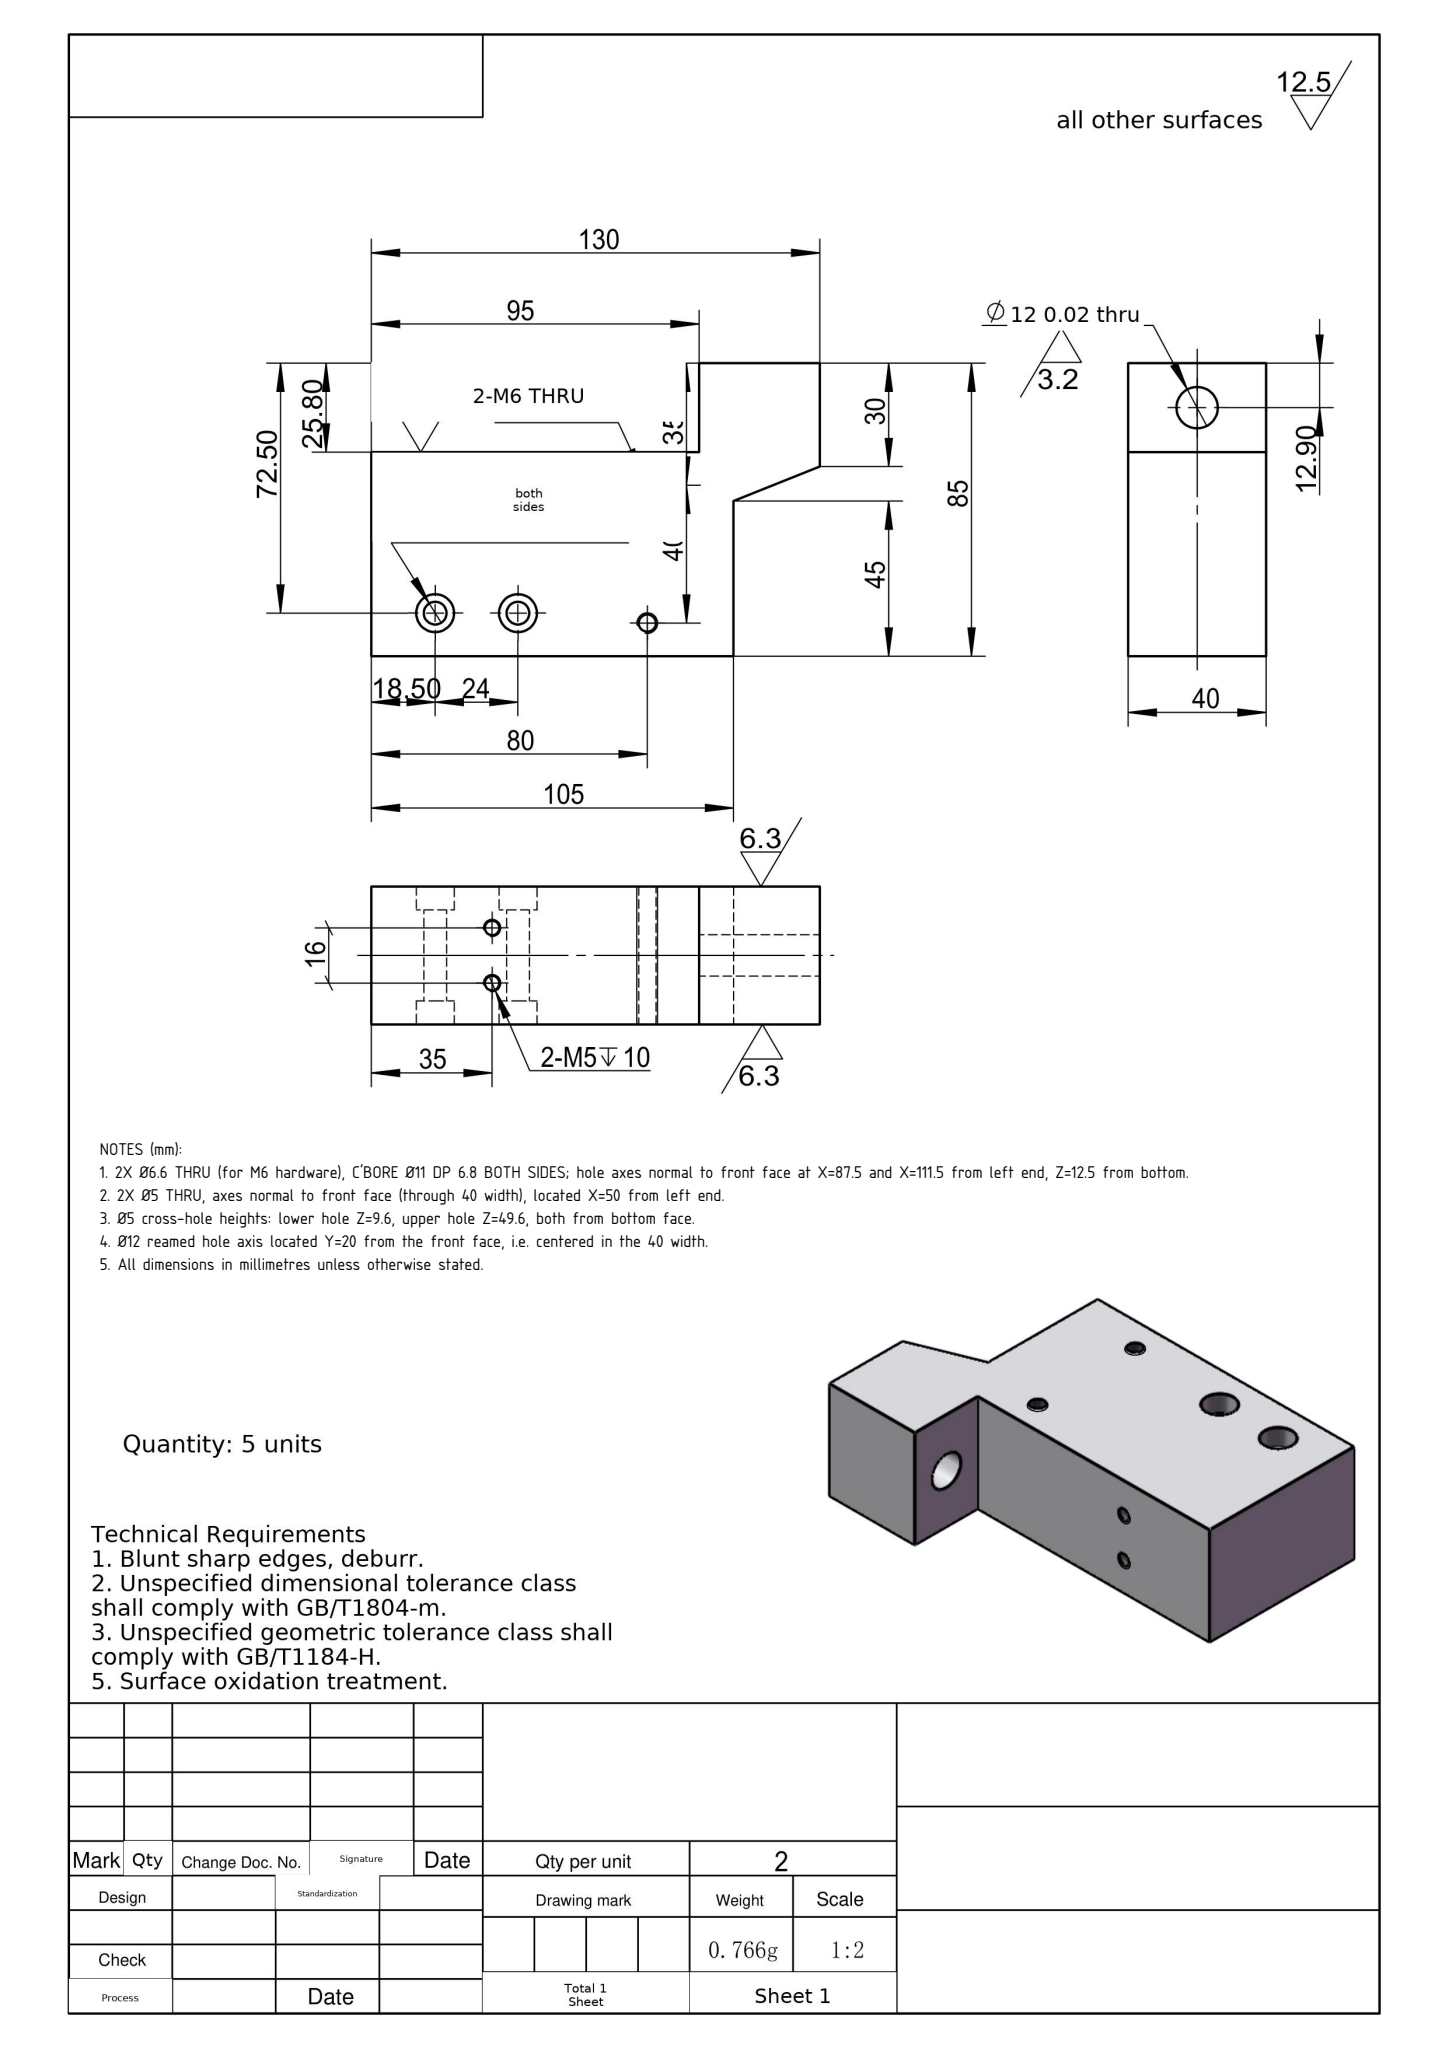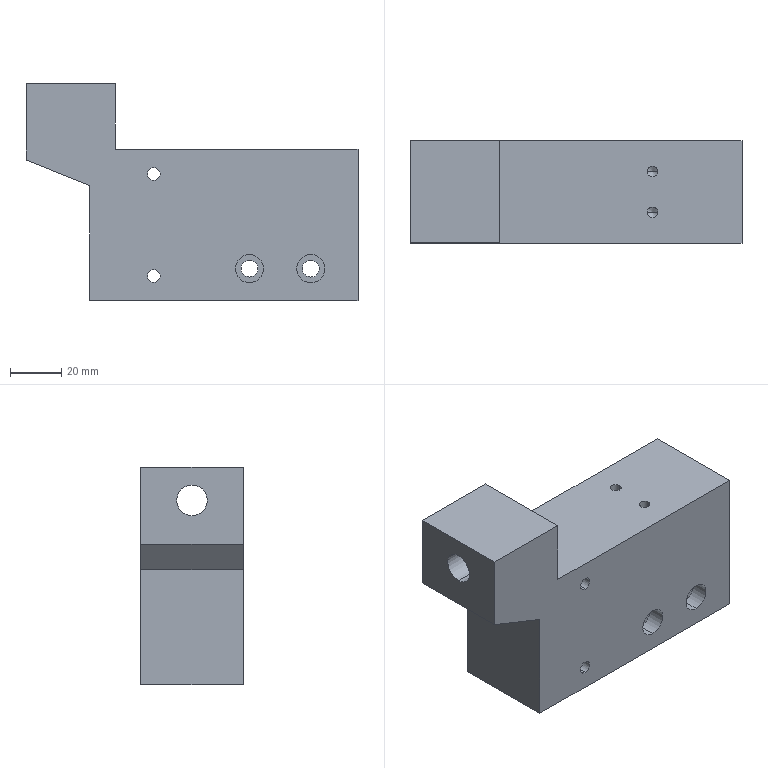Part | SolidWorks | mm | 1 solid | 40 faces | box 130 x 40 x 85 mm | volume 283640 mm3 | cylinder 22 | plane 14 | cone 4 | commonest cylinder face diameters 11 x8 5 x4 4.2 x4 6.6 x4 12 x2
Drawing notes:
2X Ø6.6 THRU (for M6 hardware), C'BORE Ø11 DP 6.8 BOTH SIDES; hole axes normal to front face at X=87.5 and X=111.5 from left end, Z=12.5 from bottom. | from the solid: cylinders: [6.6,'y',[87.5,null,12.5],26.4] and [6.6,'y',[111.5,null,12.5],26.4]; [11.0,'y',[87.5,null,12.5],6.8] and [11.0,'y',[111.5,null,12.5],6.8] (4 counterbores = both sides)
2X Ø5 THRU, axes normal to front face (through 40 width), located X=50 from left end. | from the solid: cylinders: [5.0,'y',[50.0,null,9.6],40.0] and [5.0,'y',[50.0,null,49.6],40.0]
Ø5 cross-hole heights: lower hole Z=9.6, upper hole Z=49.6, both from bottom face. | from the solid: cylinders: [5.0,'y',[50.0,null,9.6],40.0] and [5.0,'y',[50.0,null,49.6],40.0]; bbox_xyz z=85
Ø12 reamed hole axis located Y=20 from the front face, i.e. centered in the 40 width. | from the solid: cylinder [12.0,'x',[null,20.0,72.1],35.0]; bbox_xyz y=40
All dimensions in millimetres unless otherwise stated. | from the solid: STEP model facts given in mm